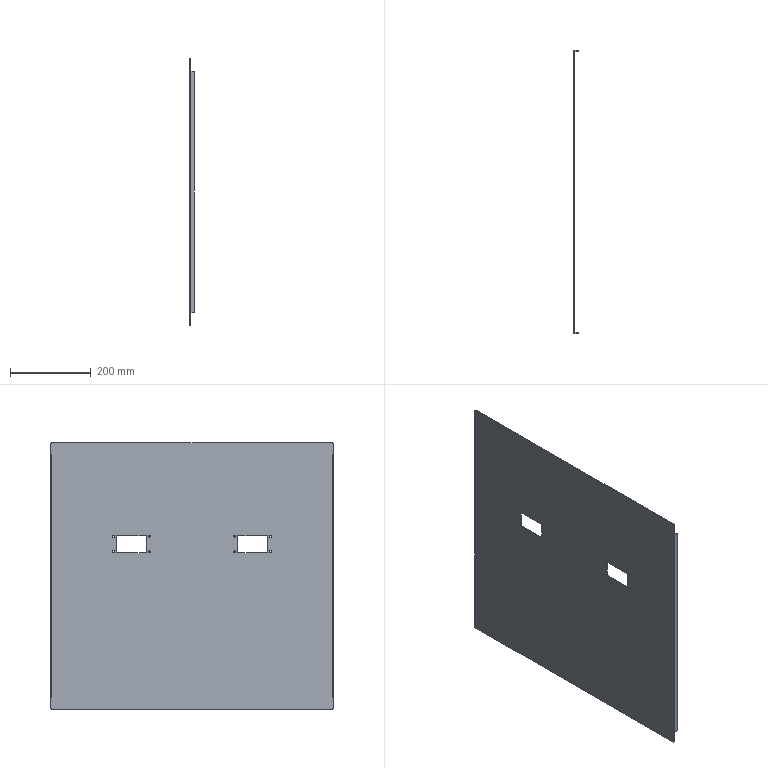Component | SolidWorks | ThreeLowRackSidePlate2-1 | 1 solid | 70 faces | volume 927871 mm3 | plane 46 | cylinder 24 | commonest cylinder face diameters 5 x16 10 x4 5.473 x2 1.473 x2 | material AISI 304